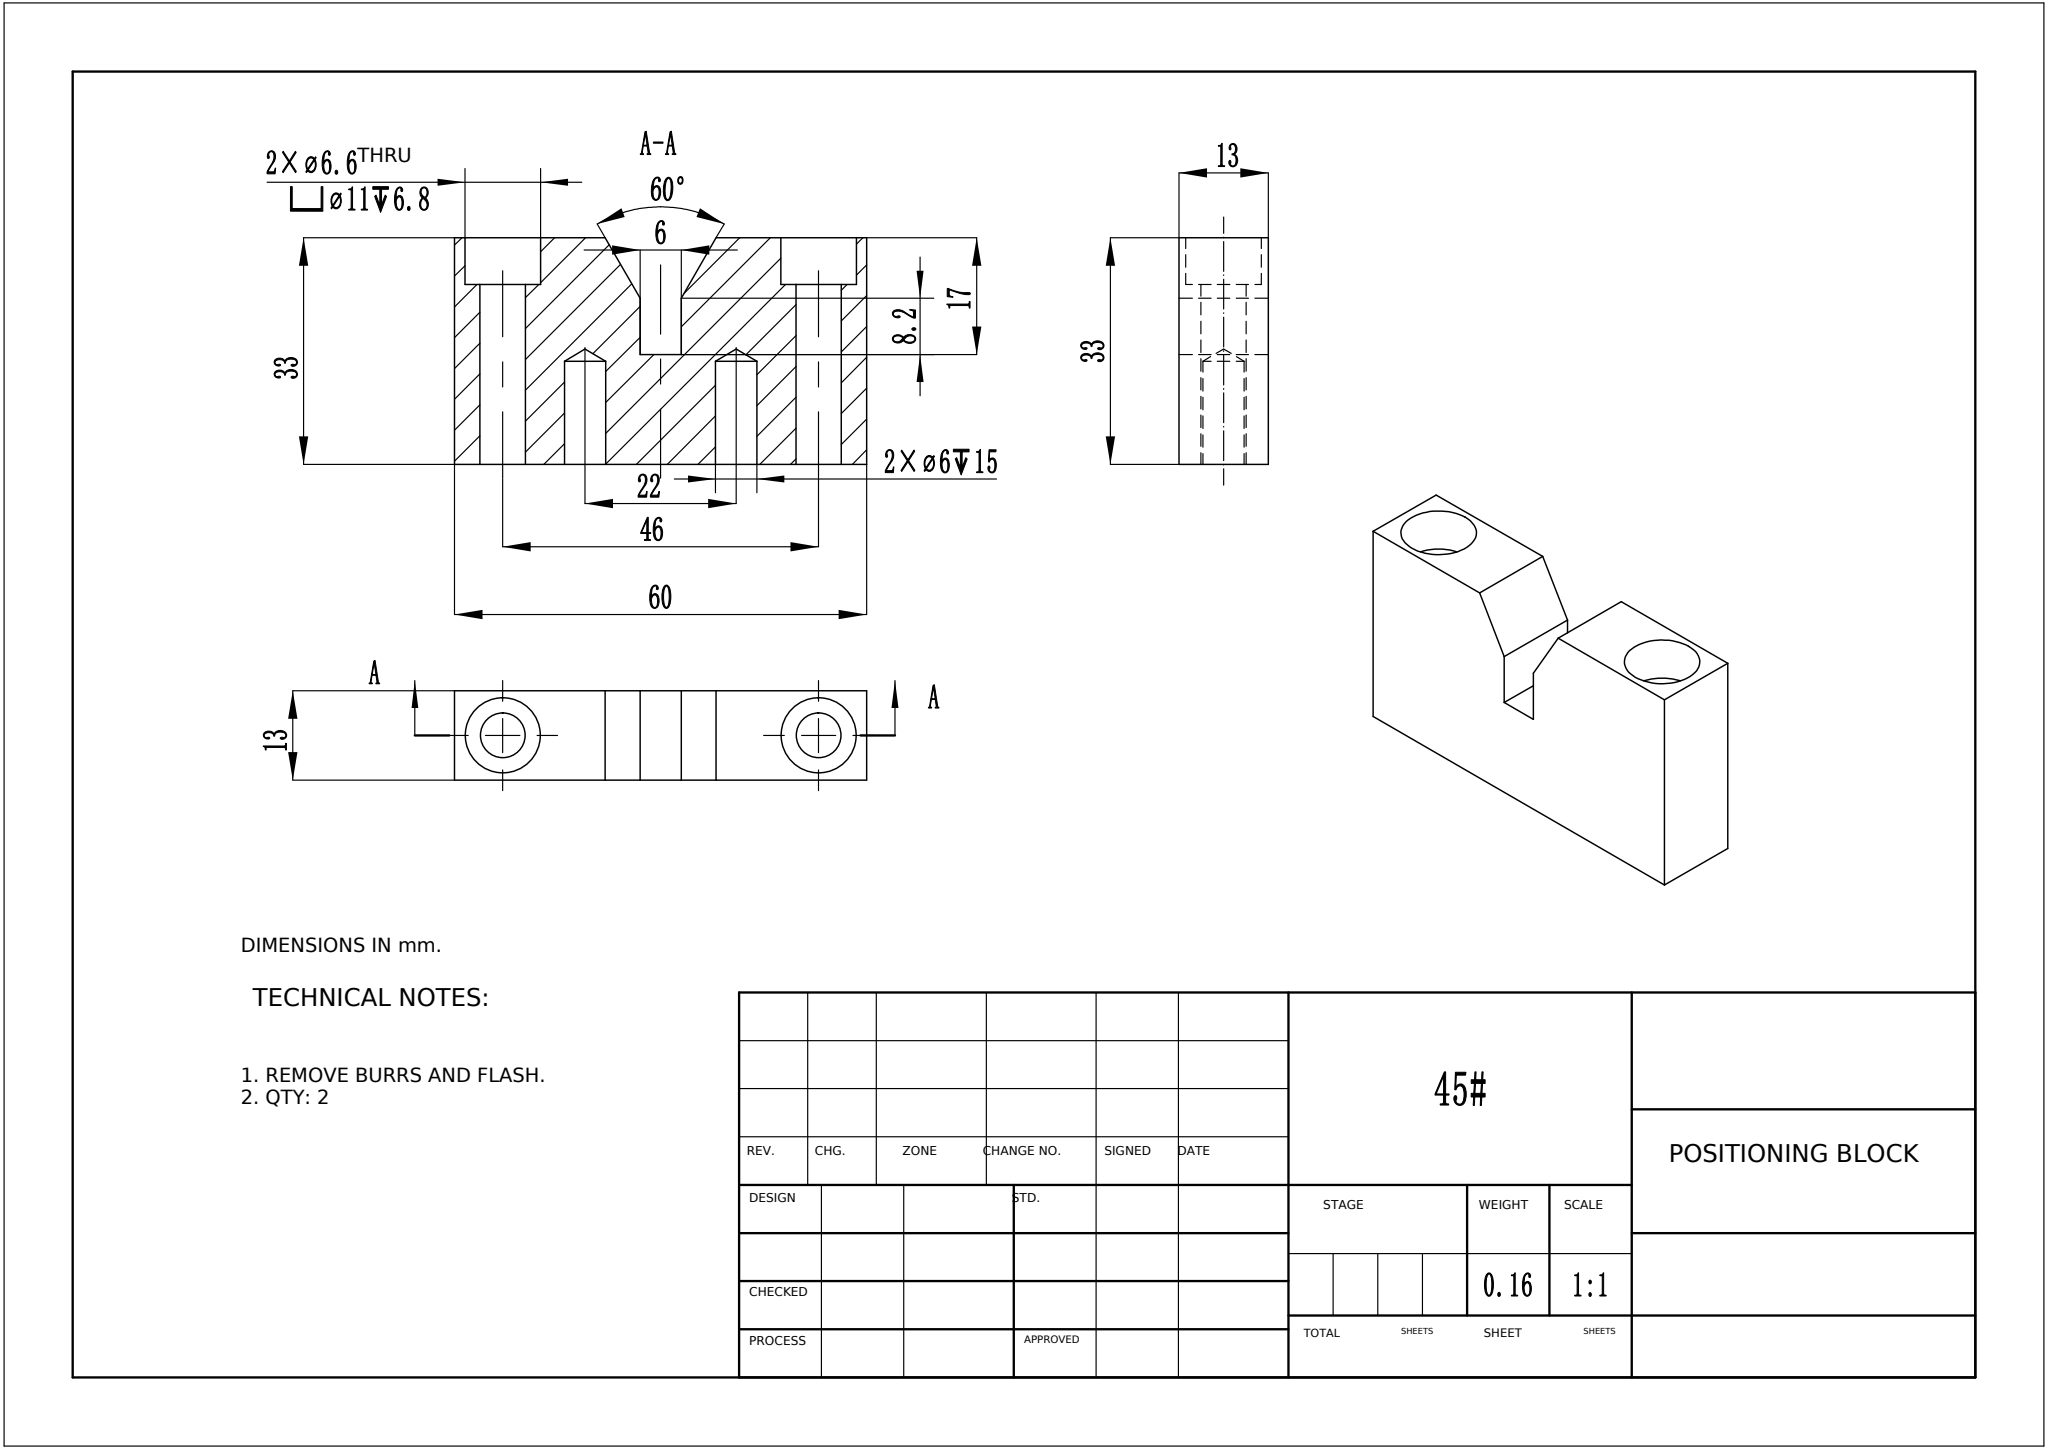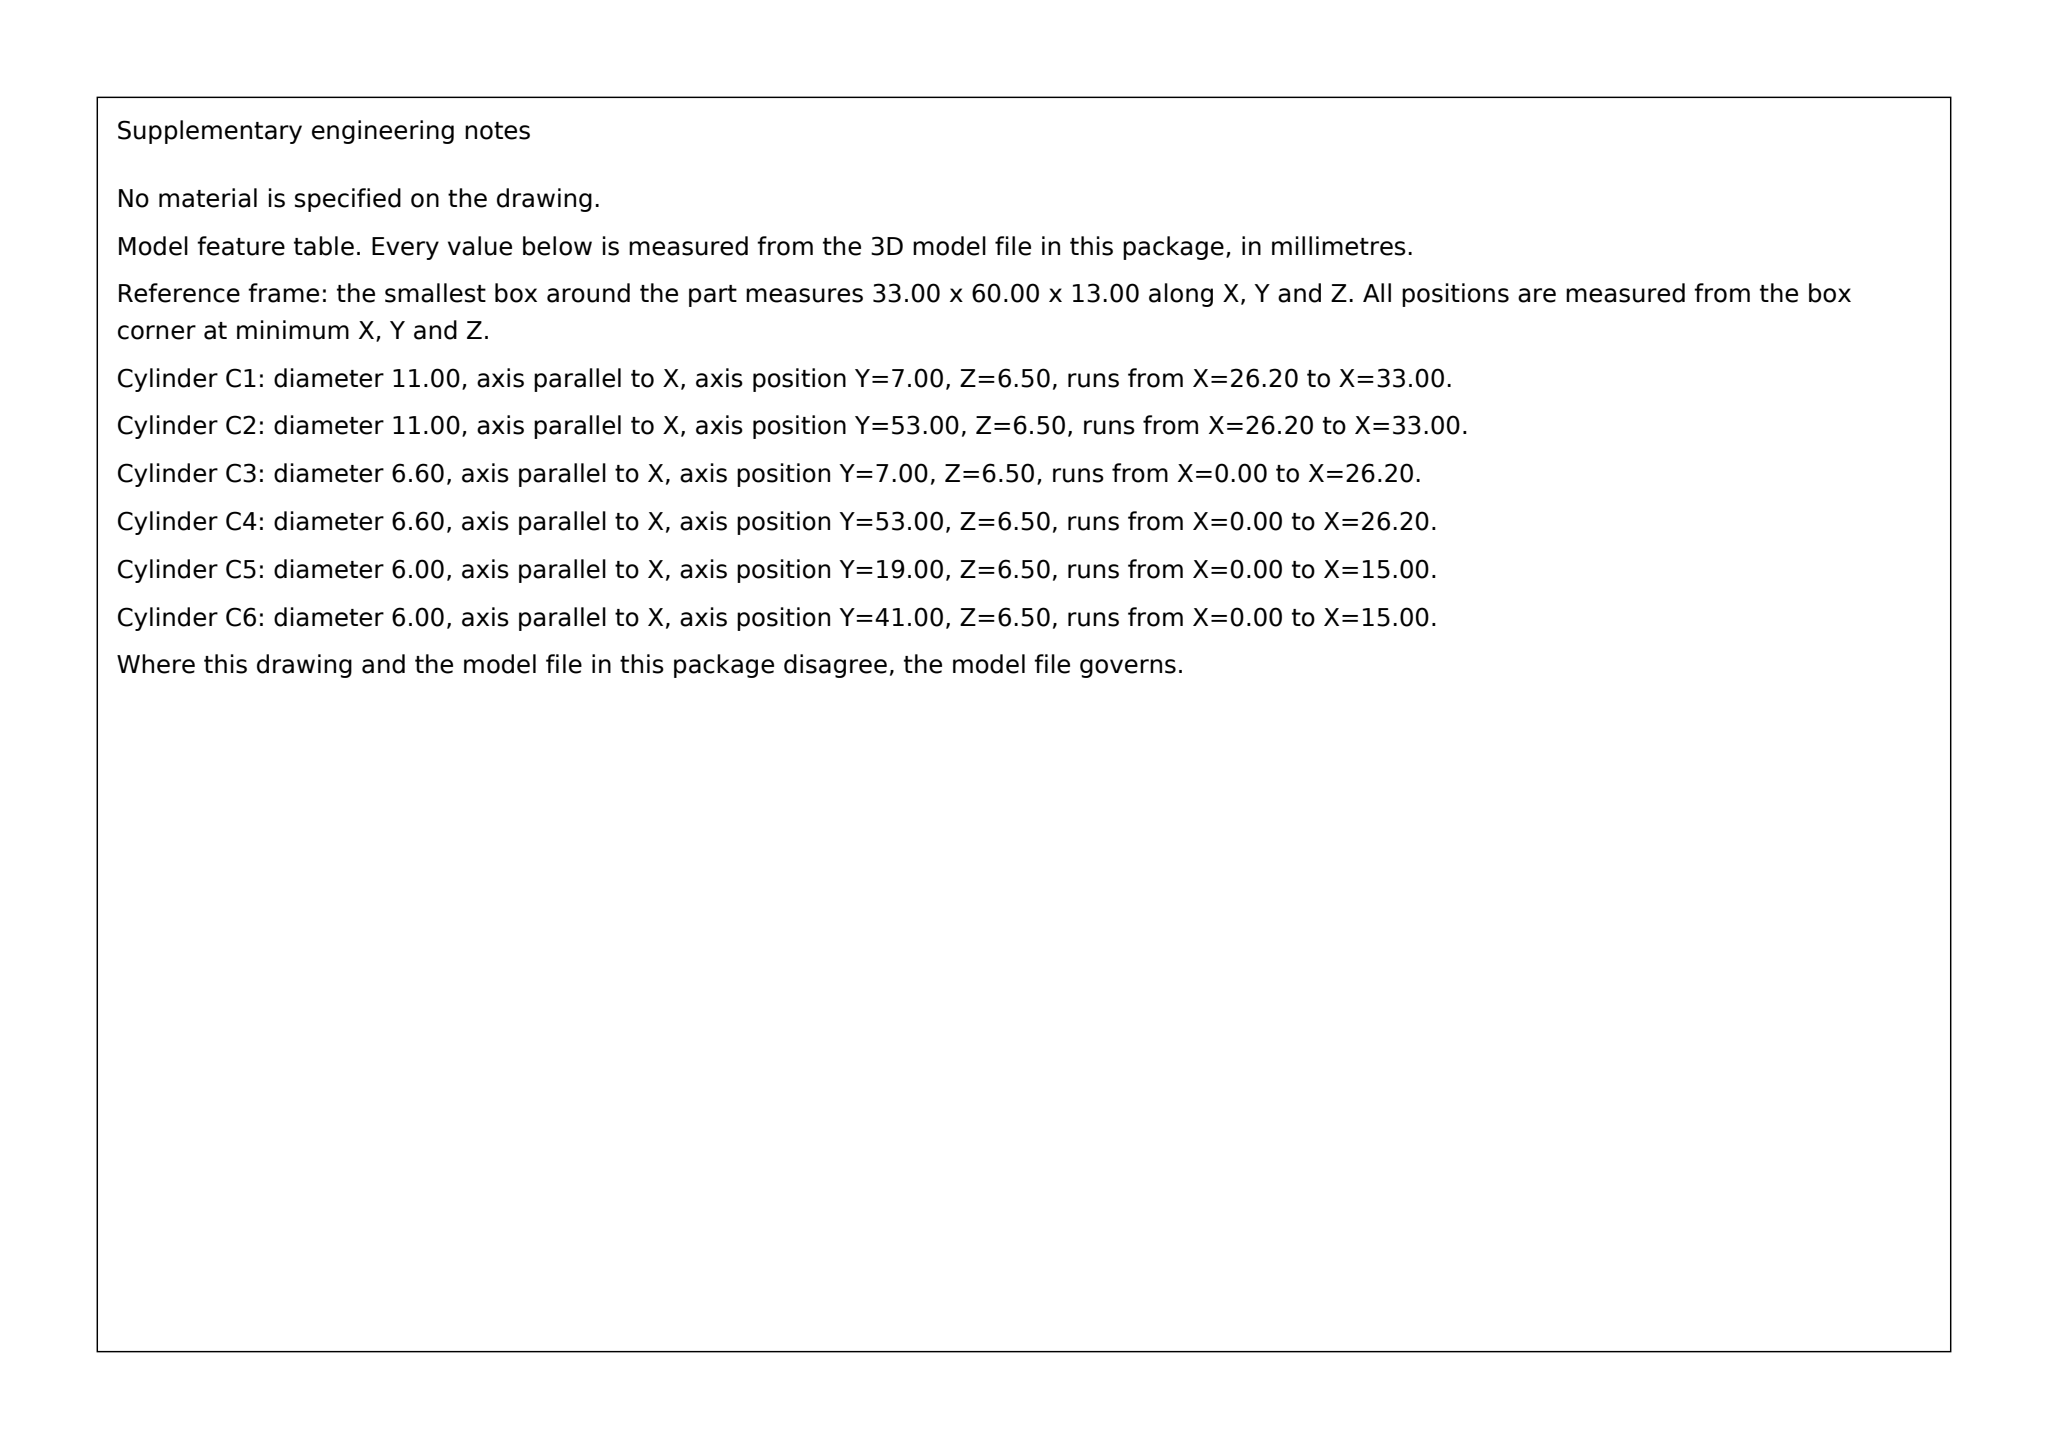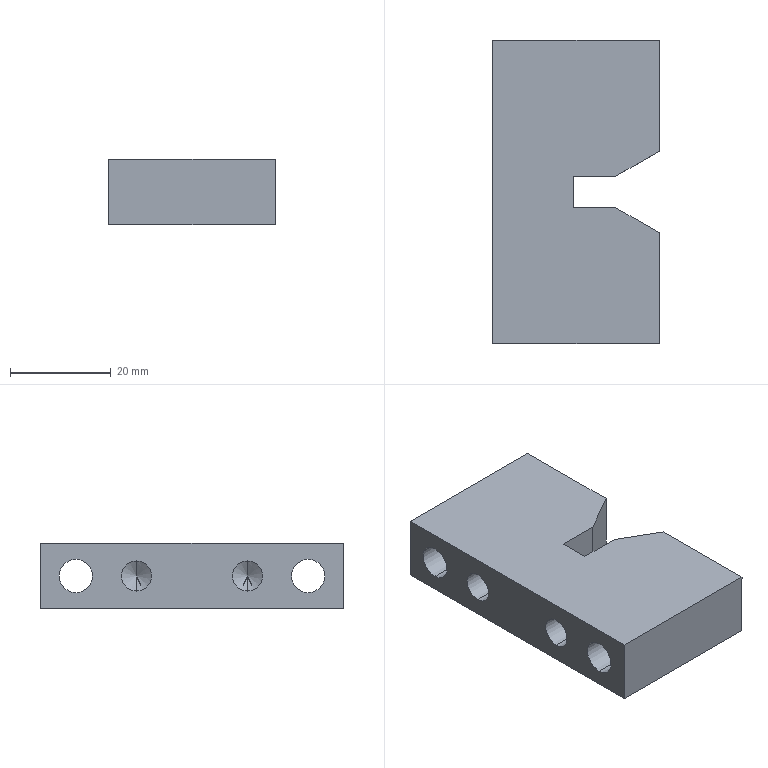Part | SolidWorks | mm | 1 solid | 30 faces | box 33 x 60 x 13 mm | volume 19865 mm3 | plane 14 | cylinder 12 | cone 4 | commonest cylinder face diameters 6 x4 11 x4 6.6 x4
build123d program:
from build123d import *

# Parameters (mm, degrees)
SKETCH1_W                                       = 100
SKETCH1_H                                       = 60
BOSS_EXTRUDE1_DEPTH                             = 50
SKETCH3_R                                       = 6.75
CUT_EXTRUDE1_DEPTH                              = 116.758
BOSS_EXTRUDE2_DEPTH                             = 156
CUT_EXTRUDE4_DEPTH                              = 180.818
SKETCH6_W                                       = 65
SKETCH6_H                                       = 60
CUT_EXTRUDE5_DEPTH                              = 63.682
BOSS_EXTRUDE4_DEPTH                             = 13
SKETCH9_W                                       = 13.769
SKETCH9_H                                       = 6
CUT_EXTRUDE6_DEPTH                              = 52.517
MOVE_FACE1_BY                                   = 10
SKETCH14_W                                      = 23.752
SKETCH14_H                                      = 71.896
CUT_EXTRUDE9_DEPTH                              = 68
M6_HEX_SOCKET_HEAD_CAP_SCREW_CBORE1_D           = 6.6
M6_HEX_SOCKET_HEAD_CAP_SCREW_CBORE1_CBORE_D     = 11
M6_HEX_SOCKET_HEAD_CAP_SCREW_CBORE1_CBORE_DEPTH = 6.8
F_6_0MM_BLIND_PIN_HOLE1_D                       = 6
F_6_0MM_BLIND_PIN_HOLE1_DEPTH                   = 15
F_6_0MM_BLIND_PIN_HOLE1_TIP                     = 1.803


with BuildPart() as part:
    # Sketch1 → Boss-Extrude1 (new body)
    with BuildSketch(Plane(origin=(0, 0, 0), x_dir=(0, 0, -1), z_dir=(1, 0, 0))):
        Rectangle(SKETCH1_W, SKETCH1_H)
    extrude(amount=BOSS_EXTRUDE1_DEPTH)

    # Sketch3 → Cut-Extrude1 (cut, through all)
    with BuildSketch(Plane.XY.offset(50)):
        with Locations((20, 0)):
            Circle(SKETCH3_R)
    extrude(amount=-CUT_EXTRUDE1_DEPTH, mode=Mode.SUBTRACT)

    # Sketch4 → Boss-Extrude2 (add)
    with BuildSketch(Plane.XY.offset(50)):
        Polygon((6.5, 0), (23, -9.526), (23, -55.864), (61.54, -55.864), (61.54, 64.895), (23, 64.895), (23, 9.526), align=None)
    extrude(amount=-BOSS_EXTRUDE2_DEPTH)

    # Sketch5 → Cut-Extrude4 (cut, through all)
    with BuildSketch(Plane(origin=(0, 0, -106), x_dir=(-1, 0, 0), z_dir=(0, 0, -1))):
        Polygon((-23, 9.526), (-23, 64.895), (-61.54, 64.895), (-61.54, -55.864), (-23, -55.864), (-23, -9.526), (-6.5, 0), align=None)
    extrude(amount=-CUT_EXTRUDE4_DEPTH, mode=Mode.SUBTRACT)

    # Sketch6 → Cut-Extrude5 (cut, through all)
    with BuildSketch(Plane(origin=(23, 0, 0), x_dir=(0, 0, -1), z_dir=(1, 0, 0))):
        with Locations((17.5, 0)):
            Rectangle(SKETCH6_W, SKETCH6_H)
    extrude(amount=-CUT_EXTRUDE5_DEPTH, mode=Mode.SUBTRACT)

    # Sketch10 → Boss-Extrude4 (add)
    with BuildSketch(Plane.XY.offset(50)):
        Polygon((23, 8.083), (9, 0), (23, -8.083), (23, -13.063), (5.064, -13.063), (5.064, 13.423), (23, 13.423), align=None)
    extrude(amount=-BOSS_EXTRUDE4_DEPTH)

    # Sketch9 → Cut-Extrude6 (cut, through all)
    with BuildSketch(Plane.XY.offset(50)):
        with Locations((12.884, 0)):
            Rectangle(SKETCH9_W, SKETCH9_H)
    extrude(amount=-CUT_EXTRUDE6_DEPTH, mode=Mode.SUBTRACT)

    # Move Face1: a face moved outward by 10.0
    extrude(part.faces().sort_by_distance((0, 0, 32.5))[0], amount=MOVE_FACE1_BY, dir=(-1, 0, 0))

    # Sketch14 → Cut-Extrude9 (cut, through all)
    with BuildSketch(Plane(origin=(23, 0, 0), x_dir=(0, 0, -1), z_dir=(1, 0, 0))):
        with Locations((-25.124, 2.799)):
            Rectangle(SKETCH14_W, SKETCH14_H)
    extrude(amount=-CUT_EXTRUDE9_DEPTH, mode=Mode.SUBTRACT)

    # M6 Hex Socket Head Cap Screw CBORE1 (through all)
    with Locations(Plane(origin=(23, 0, 0), x_dir=(0, 0, -1), z_dir=(1, 0, 0))):
        with Locations((-43.5, 23), (-43.5, -23)):
            CounterBoreHole(M6_HEX_SOCKET_HEAD_CAP_SCREW_CBORE1_D / 2, M6_HEX_SOCKET_HEAD_CAP_SCREW_CBORE1_CBORE_D / 2, M6_HEX_SOCKET_HEAD_CAP_SCREW_CBORE1_CBORE_DEPTH)

    # 6.0mm Blind Pin Hole1
    with Locations(Plane.ZY.offset(10)):
        with Locations((43.5, 11), (43.5, -11)):
            Hole(F_6_0MM_BLIND_PIN_HOLE1_D / 2, depth=F_6_0MM_BLIND_PIN_HOLE1_DEPTH)
            with Locations((0, 0, -(F_6_0MM_BLIND_PIN_HOLE1_DEPTH + F_6_0MM_BLIND_PIN_HOLE1_TIP / 2))):  # 118° drill point
                Cone(0, F_6_0MM_BLIND_PIN_HOLE1_D / 2, F_6_0MM_BLIND_PIN_HOLE1_TIP, mode=Mode.SUBTRACT)


solid = part.part
STEP:
#1=CARTESIAN_POINT('',(5.,11.,40.5));
#2=VERTEX_POINT('',#1);
#3=CARTESIAN_POINT('',(5.,11.,46.5));
#4=VERTEX_POINT('',#3);
#5=CARTESIAN_POINT('',(5.,11.,43.5));
#6=DIRECTION('',(-1.,0.,0.));
#7=DIRECTION('',(0.,0.,1.));
#8=AXIS2_PLACEMENT_3D('',#5,#6,#7);
#9=CIRCLE('',#8,3.);
#10=EDGE_CURVE('',#2,#4,#9,.T.);
#11=ORIENTED_EDGE('',*,*,#10,.F.);
#12=CARTESIAN_POINT('',(-10.,11.,40.5));
#13=VERTEX_POINT('',#12);
#14=CARTESIAN_POINT('',(-10.,11.,40.5));
#15=DIRECTION('',(-1.,0.,0.));
#16=VECTOR('',#15,1000.);
#17=LINE('',#14,#16);
#18=EDGE_CURVE('',#2,#13,#17,.T.);
#19=ORIENTED_EDGE('',*,*,#18,.T.);
#20=CARTESIAN_POINT('',(-10.,11.,46.5));
#21=VERTEX_POINT('',#20);
#22=CARTESIAN_POINT('',(-10.,11.,43.5));
#23=DIRECTION('',(-1.,0.,0.));
#24=DIRECTION('',(0.,0.,1.));
#25=AXIS2_PLACEMENT_3D('',#22,#23,#24);
#26=CIRCLE('',#25,3.);
#27=EDGE_CURVE('',#13,#21,#26,.T.);
#28=ORIENTED_EDGE('',*,*,#27,.T.);
#29=CARTESIAN_POINT('',(-10.,11.,46.5));
#30=DIRECTION('',(-1.,0.,0.));
#31=VECTOR('',#30,1000.);
#32=LINE('',#29,#31);
#33=EDGE_CURVE('',#4,#21,#32,.T.);
#34=ORIENTED_EDGE('',*,*,#33,.F.);
#35=EDGE_LOOP('',(#11,#19,#28,#34));
#36=FACE_OUTER_BOUND('',#35,.T.);
#37=CARTESIAN_POINT('',(-10.,11.,43.5));
#38=DIRECTION('',(-1.,0.,0.));
#39=DIRECTION('',(0.,0.,1.));
#40=AXIS2_PLACEMENT_3D('',#37,#38,#39);
#41=CYLINDRICAL_SURFACE('',#40,3.);
#42=ADVANCED_FACE('',(#36),#41,.F.);
#43=CARTESIAN_POINT('',(6.803,11.,43.5));
#44=VERTEX_POINT('',#43);
#45=CARTESIAN_POINT('',(5.,11.,46.5));
#46=DIRECTION('',(-0.515,0.,0.8572));
#47=VECTOR('',#46,1000.);
#48=LINE('',#45,#47);
#49=EDGE_CURVE('',#44,#4,#48,.T.);
#50=ORIENTED_EDGE('',*,*,#49,.F.);
#51=CARTESIAN_POINT('',(5.,11.,40.5));
#52=DIRECTION('',(-0.515,0.,-0.8572));
#53=VECTOR('',#52,1000.);
#54=LINE('',#51,#53);
#55=EDGE_CURVE('',#44,#2,#54,.T.);
#56=ORIENTED_EDGE('',*,*,#55,.T.);
#57=ORIENTED_EDGE('',*,*,#10,.T.);
#58=EDGE_LOOP('',(#50,#56,#57));
#59=FACE_OUTER_BOUND('',#58,.T.);
#60=CARTESIAN_POINT('',(5.,11.,43.5));
#61=DIRECTION('',(-1.,0.,0.));
#62=DIRECTION('',(0.,0.,1.));
#63=AXIS2_PLACEMENT_3D('',#60,#61,#62);
#64=CONICAL_SURFACE('',#63,3.,1.03);
#65=ADVANCED_FACE('',(#59),#64,.F.);
#66=CARTESIAN_POINT('',(5.,-11.,40.5));
#67=VERTEX_POINT('',#66);
#68=CARTESIAN_POINT('',(5.,-11.,46.5));
#69=VERTEX_POINT('',#68);
#70=CARTESIAN_POINT('',(5.,-11.,43.5));
#71=DIRECTION('',(-1.,0.,0.));
#72=DIRECTION('',(0.,0.,1.));
#73=AXIS2_PLACEMENT_3D('',#70,#71,#72);
#74=CIRCLE('',#73,3.);
#75=EDGE_CURVE('',#67,#69,#74,.T.);
#76=ORIENTED_EDGE('',*,*,#75,.F.);
#77=CARTESIAN_POINT('',(-10.,-11.,40.5));
#78=VERTEX_POINT('',#77);
#79=CARTESIAN_POINT('',(-10.,-11.,40.5));
#80=DIRECTION('',(-1.,0.,0.));
#81=VECTOR('',#80,1000.);
#82=LINE('',#79,#81);
#83=EDGE_CURVE('',#67,#78,#82,.T.);
#84=ORIENTED_EDGE('',*,*,#83,.T.);
#85=CARTESIAN_POINT('',(-10.,-11.,46.5));
#86=VERTEX_POINT('',#85);
#87=CARTESIAN_POINT('',(-10.,-11.,43.5));
#88=DIRECTION('',(-1.,0.,0.));
#89=DIRECTION('',(0.,0.,1.));
#90=AXIS2_PLACEMENT_3D('',#87,#88,#89);
#91=CIRCLE('',#90,3.);
#92=EDGE_CURVE('',#78,#86,#91,.T.);
#93=ORIENTED_EDGE('',*,*,#92,.T.);
#94=CARTESIAN_POINT('',(-10.,-11.,46.5));
#95=DIRECTION('',(-1.,0.,0.));
#96=VECTOR('',#95,1000.);
#97=LINE('',#94,#96);
#98=EDGE_CURVE('',#69,#86,#97,.T.);
#99=ORIENTED_EDGE('',*,*,#98,.F.);
#100=EDGE_LOOP('',(#76,#84,#93,#99));
#101=FACE_OUTER_BOUND('',#100,.T.);
#102=CARTESIAN_POINT('',(-10.,-11.,43.5));
#103=DIRECTION('',(-1.,0.,0.));
#104=DIRECTION('',(0.,0.,1.));
#105=AXIS2_PLACEMENT_3D('',#102,#103,#104);
#106=CYLINDRICAL_SURFACE('',#105,3.);
#107=ADVANCED_FACE('',(#101),#106,.F.);
#108=CARTESIAN_POINT('',(6.803,-11.,43.5));
#109=VERTEX_POINT('',#108);
#110=CARTESIAN_POINT('',(5.,-11.,46.5));
#111=DIRECTION('',(-0.515,0.,0.8572));
#112=VECTOR('',#111,1000.);
#113=LINE('',#110,#112);
#114=EDGE_CURVE('',#109,#69,#113,.T.);
#115=ORIENTED_EDGE('',*,*,#114,.F.);
#116=CARTESIAN_POINT('',(5.,-11.,40.5));
#117=DIRECTION('',(-0.515,0.,-0.8572));
#118=VECTOR('',#117,1000.);
#119=LINE('',#116,#118);
#120=EDGE_CURVE('',#109,#67,#119,.T.);
#121=ORIENTED_EDGE('',*,*,#120,.T.);
#122=ORIENTED_EDGE('',*,*,#75,.T.);
#123=EDGE_LOOP('',(#115,#121,#122));
#124=FACE_OUTER_BOUND('',#123,.T.);
#125=CARTESIAN_POINT('',(5.,-11.,43.5));
#126=DIRECTION('',(-1.,0.,0.));
#127=DIRECTION('',(0.,0.,1.));
#128=AXIS2_PLACEMENT_3D('',#125,#126,#127);
#129=CONICAL_SURFACE('',#128,3.,1.03);
#130=ADVANCED_FACE('',(#124),#129,.F.);
#131=CARTESIAN_POINT('',(16.2,23.,49.));
#132=VERTEX_POINT('',#131);
#133=CARTESIAN_POINT('',(16.2,23.,38.));
#134=VERTEX_POINT('',#133);
#135=CARTESIAN_POINT('',(16.2,23.,43.5));
#136=DIRECTION('',(1.,0.,0.));
#137=DIRECTION('',(0.,0.,-1.));
#138=AXIS2_PLACEMENT_3D('',#135,#136,#137);
#139=CIRCLE('',#138,5.5);
#140=EDGE_CURVE('',#132,#134,#139,.T.);
#141=ORIENTED_EDGE('',*,*,#140,.F.);
#142=CARTESIAN_POINT('',(23.,23.,49.));
#143=VERTEX_POINT('',#142);
#144=CARTESIAN_POINT('',(23.,23.,49.));
#145=DIRECTION('',(1.,0.,0.));
#146=VECTOR('',#145,1000.);
#147=LINE('',#144,#146);
#148=EDGE_CURVE('',#132,#143,#147,.T.);
#149=ORIENTED_EDGE('',*,*,#148,.T.);
#150=CARTESIAN_POINT('',(23.,23.,38.));
#151=VERTEX_POINT('',#150);
#152=CARTESIAN_POINT('',(23.,23.,43.5));
#153=DIRECTION('',(1.,0.,0.));
#154=DIRECTION('',(0.,0.,-1.));
#155=AXIS2_PLACEMENT_3D('',#152,#153,#154);
#156=CIRCLE('',#155,5.5);
#157=EDGE_CURVE('',#143,#151,#156,.T.);
#158=ORIENTED_EDGE('',*,*,#157,.T.);
#159=CARTESIAN_POINT('',(23.,23.,38.));
#160=DIRECTION('',(1.,0.,0.));
#161=VECTOR('',#160,1000.);
#162=LINE('',#159,#161);
#163=EDGE_CURVE('',#134,#151,#162,.T.);
#164=ORIENTED_EDGE('',*,*,#163,.F.);
#165=EDGE_LOOP('',(#141,#149,#158,#164));
#166=FACE_OUTER_BOUND('',#165,.T.);
#167=CARTESIAN_POINT('',(23.,23.,43.5));
#168=DIRECTION('',(1.,0.,0.));
#169=DIRECTION('',(0.,0.,-1.));
#170=AXIS2_PLACEMENT_3D('',#167,#168,#169);
#171=CYLINDRICAL_SURFACE('',#170,5.5);
#172=ADVANCED_FACE('',(#166),#171,.F.);
#173=CARTESIAN_POINT('',(-10.,23.,46.8));
#174=VERTEX_POINT('',#173);
#175=CARTESIAN_POINT('',(-10.,23.,40.2));
#176=VERTEX_POINT('',#175);
#177=CARTESIAN_POINT('',(-10.,23.,43.5));
#178=DIRECTION('',(1.,0.,0.));
#179=DIRECTION('',(0.,0.,-1.));
#180=AXIS2_PLACEMENT_3D('',#177,#178,#179);
#181=CIRCLE('',#180,3.3);
#182=EDGE_CURVE('',#174,#176,#181,.T.);
#183=ORIENTED_EDGE('',*,*,#182,.F.);
#184=CARTESIAN_POINT('',(16.2,23.,46.8));
#185=VERTEX_POINT('',#184);
#186=CARTESIAN_POINT('',(23.,23.,46.8));
#187=DIRECTION('',(1.,0.,0.));
#188=VECTOR('',#187,1000.);
#189=LINE('',#186,#188);
#190=EDGE_CURVE('',#174,#185,#189,.T.);
#191=ORIENTED_EDGE('',*,*,#190,.T.);
#192=CARTESIAN_POINT('',(16.2,23.,40.2));
#193=VERTEX_POINT('',#192);
#194=CARTESIAN_POINT('',(16.2,23.,43.5));
#195=DIRECTION('',(1.,0.,0.));
#196=DIRECTION('',(0.,0.,-1.));
#197=AXIS2_PLACEMENT_3D('',#194,#195,#196);
#198=CIRCLE('',#197,3.3);
#199=EDGE_CURVE('',#185,#193,#198,.T.);
#200=ORIENTED_EDGE('',*,*,#199,.T.);
#201=CARTESIAN_POINT('',(23.,23.,40.2));
#202=DIRECTION('',(1.,0.,0.));
#203=VECTOR('',#202,1000.);
#204=LINE('',#201,#203);
#205=EDGE_CURVE('',#176,#193,#204,.T.);
#206=ORIENTED_EDGE('',*,*,#205,.F.);
#207=EDGE_LOOP('',(#183,#191,#200,#206));
#208=FACE_OUTER_BOUND('',#207,.T.);
#209=CARTESIAN_POINT('',(23.,23.,43.5));
#210=DIRECTION('',(1.,0.,0.));
#211=DIRECTION('',(0.,0.,-1.));
#212=AXIS2_PLACEMENT_3D('',#209,#210,#211);
#213=CYLINDRICAL_SURFACE('',#212,3.3);
#214=ADVANCED_FACE('',(#208),#213,.F.);
#215=CARTESIAN_POINT('',(16.2,-23.,49.));
#216=VERTEX_POINT('',#215);
#217=CARTESIAN_POINT('',(16.2,-23.,38.));
#218=VERTEX_POINT('',#217);
#219=CARTESIAN_POINT('',(16.2,-23.,43.5));
#220=DIRECTION('',(1.,0.,0.));
#221=DIRECTION('',(0.,0.,-1.));
#222=AXIS2_PLACEMENT_3D('',#219,#220,#221);
#223=CIRCLE('',#222,5.5);
#224=EDGE_CURVE('',#216,#218,#223,.T.);
#225=ORIENTED_EDGE('',*,*,#224,.F.);
#226=CARTESIAN_POINT('',(23.,-23.,49.));
#227=VERTEX_POINT('',#226);
#228=CARTESIAN_POINT('',(23.,-23.,49.));
#229=DIRECTION('',(1.,0.,0.));
#230=VECTOR('',#229,1000.);
#231=LINE('',#228,#230);
#232=EDGE_CURVE('',#216,#227,#231,.T.);
#233=ORIENTED_EDGE('',*,*,#232,.T.);
#234=CARTESIAN_POINT('',(23.,-23.,38.));
#235=VERTEX_POINT('',#234);
#236=CARTESIAN_POINT('',(23.,-23.,43.5));
#237=DIRECTION('',(1.,0.,0.));
#238=DIRECTION('',(0.,0.,-1.));
#239=AXIS2_PLACEMENT_3D('',#236,#237,#238);
#240=CIRCLE('',#239,5.5);
#241=EDGE_CURVE('',#227,#235,#240,.T.);
#242=ORIENTED_EDGE('',*,*,#241,.T.);
#243=CARTESIAN_POINT('',(23.,-23.,38.));
#244=DIRECTION('',(1.,0.,0.));
#245=VECTOR('',#244,1000.);
#246=LINE('',#243,#245);
#247=EDGE_CURVE('',#218,#235,#246,.T.);
#248=ORIENTED_EDGE('',*,*,#247,.F.);
#249=EDGE_LOOP('',(#225,#233,#242,#248));
#250=FACE_OUTER_BOUND('',#249,.T.);
#251=CARTESIAN_POINT('',(23.,-23.,43.5));
#252=DIRECTION('',(1.,0.,0.));
#253=DIRECTION('',(0.,0.,-1.));
#254=AXIS2_PLACEMENT_3D('',#251,#252,#253);
#255=CYLINDRICAL_SURFACE('',#254,5.5);
#256=ADVANCED_FACE('',(#250),#255,.F.);
#257=CARTESIAN_POINT('',(-10.,-23.,46.8));
#258=VERTEX_POINT('',#257);
#259=CARTESIAN_POINT('',(-10.,-23.,40.2));
#260=VERTEX_POINT('',#259);
#261=CARTESIAN_POINT('',(-10.,-23.,43.5));
#262=DIRECTION('',(1.,0.,0.));
#263=DIRECTION('',(0.,0.,-1.));
#264=AXIS2_PLACEMENT_3D('',#261,#262,#263);
#265=CIRCLE('',#264,3.3);
#266=EDGE_CURVE('',#258,#260,#265,.T.);
#267=ORIENTED_EDGE('',*,*,#266,.F.);
#268=CARTESIAN_POINT('',(16.2,-23.,46.8));
#269=VERTEX_POINT('',#268);
#270=CARTESIAN_POINT('',(23.,-23.,46.8));
#271=DIRECTION('',(1.,0.,0.));
#272=VECTOR('',#271,1000.);
#273=LINE('',#270,#272);
#274=EDGE_CURVE('',#258,#269,#273,.T.);
#275=ORIENTED_EDGE('',*,*,#274,.T.);
#276=CARTESIAN_POINT('',(16.2,-23.,40.2));
#277=VERTEX_POINT('',#276);
#278=CARTESIAN_POINT('',(16.2,-23.,43.5));
#279=DIRECTION('',(1.,0.,0.));
#280=DIRECTION('',(0.,0.,-1.));
#281=AXIS2_PLACEMENT_3D('',#278,#279,#280);
#282=CIRCLE('',#281,3.3);
#283=EDGE_CURVE('',#269,#277,#282,.T.);
#284=ORIENTED_EDGE('',*,*,#283,.T.);
#285=CARTESIAN_POINT('',(23.,-23.,40.2));
#286=DIRECTION('',(1.,0.,0.));
#287=VECTOR('',#286,1000.);
#288=LINE('',#285,#287);
#289=EDGE_CURVE('',#260,#277,#288,.T.);
#290=ORIENTED_EDGE('',*,*,#289,.F.);
#291=EDGE_LOOP('',(#267,#275,#284,#290));
#292=FACE_OUTER_BOUND('',#291,.T.);
#293=CARTESIAN_POINT('',(23.,-23.,43.5));
#294=DIRECTION('',(1.,0.,0.));
#295=DIRECTION('',(0.,0.,-1.));
#296=AXIS2_PLACEMENT_3D('',#293,#294,#295);
#297=CYLINDRICAL_SURFACE('',#296,3.3);
#298=ADVANCED_FACE('',(#292),#297,.F.);
#299=CARTESIAN_POINT('',(23.,30.,37.));
#300=VERTEX_POINT('',#299);
#301=CARTESIAN_POINT('',(23.,30.,50.));
#302=VERTEX_POINT('',#301);
#303=CARTESIAN_POINT('',(23.,30.,-50.));
#304=DIRECTION('',(0.,-0.,1.));
#305=VECTOR('',#304,1000.);
#306=LINE('',#303,#305);
#307=EDGE_CURVE('',#300,#302,#306,.T.);
#308=ORIENTED_EDGE('',*,*,#307,.F.);
#309=CARTESIAN_POINT('',(-10.,30.,37.));
#310=VERTEX_POINT('',#309);
#311=CARTESIAN_POINT('',(50.,30.,37.));
#312=DIRECTION('',(-1.,0.,0.));
#313=VECTOR('',#312,1000.);
#314=LINE('',#311,#313);
#315=EDGE_CURVE('',#300,#310,#314,.T.);
#316=ORIENTED_EDGE('',*,*,#315,.T.);
#317=CARTESIAN_POINT('',(-10.,30.,50.));
#318=VERTEX_POINT('',#317);
#319=CARTESIAN_POINT('',(-10.,30.,-50.));
#320=DIRECTION('',(0.,-0.,1.));
#321=VECTOR('',#320,1000.);
#322=LINE('',#319,#321);
#323=EDGE_CURVE('',#310,#318,#322,.T.);
#324=ORIENTED_EDGE('',*,*,#323,.T.);
#325=CARTESIAN_POINT('',(50.,30.,50.));
#326=DIRECTION('',(-1.,0.,0.));
#327=VECTOR('',#326,1000.);
#328=LINE('',#325,#327);
#329=EDGE_CURVE('',#302,#318,#328,.T.);
#330=ORIENTED_EDGE('',*,*,#329,.F.);
#331=EDGE_LOOP('',(#308,#316,#324,#330));
#332=FACE_OUTER_BOUND('',#331,.T.);
#333=CARTESIAN_POINT('',(50.,30.,-50.));
#334=DIRECTION('',(0.,-1.,-0.));
#335=DIRECTION('',(0.,0.,-1.));
#336=AXIS2_PLACEMENT_3D('',#333,#334,#335);
#337=PLANE('',#336);
#338=ADVANCED_FACE('',(#332),#337,.F.);
#339=CARTESIAN_POINT('',(6.,3.,50.));
#340=VERTEX_POINT('',#339);
#341=CARTESIAN_POINT('',(6.,-3.,50.));
#342=VERTEX_POINT('',#341);
#343=CARTESIAN_POINT('',(6.,-3.,50.));
#344=DIRECTION('',(0.,-1.,0.));
#345=VECTOR('',#344,1000.);
#346=LINE('',#343,#345);
#347=EDGE_CURVE('',#340,#342,#346,.T.);
#348=ORIENTED_EDGE('',*,*,#347,.F.);
#349=CARTESIAN_POINT('',(14.196,3.,50.));
#350=VERTEX_POINT('',#349);
#351=CARTESIAN_POINT('',(19.769,3.,50.));
#352=DIRECTION('',(-1.,-0.,0.));
#353=VECTOR('',#352,1000.);
#354=LINE('',#351,#353);
#355=EDGE_CURVE('',#350,#340,#354,.T.);
#356=ORIENTED_EDGE('',*,*,#355,.F.);
#357=CARTESIAN_POINT('',(23.,8.083,50.));
#358=VERTEX_POINT('',#357);
#359=CARTESIAN_POINT('',(23.,8.083,50.));
#360=DIRECTION('',(0.866,0.5,0.));
#361=VECTOR('',#360,1000.);
#362=LINE('',#359,#361);
#363=EDGE_CURVE('',#350,#358,#362,.T.);
#364=ORIENTED_EDGE('',*,*,#363,.T.);
#365=CARTESIAN_POINT('',(23.,9.526,50.));
#366=DIRECTION('',(0.,1.,0.));
#367=VECTOR('',#366,1000.);
#368=LINE('',#365,#367);
#369=EDGE_CURVE('',#358,#302,#368,.T.);
#370=ORIENTED_EDGE('',*,*,#369,.T.);
#371=ORIENTED_EDGE('',*,*,#329,.T.);
#372=CARTESIAN_POINT('',(-10.,-30.,50.));
#373=VERTEX_POINT('',#372);
#374=CARTESIAN_POINT('',(-10.,-30.,50.));
#375=DIRECTION('',(0.,-1.,0.));
#376=VECTOR('',#375,1000.);
#377=LINE('',#374,#376);
#378=EDGE_CURVE('',#318,#373,#377,.T.);
#379=ORIENTED_EDGE('',*,*,#378,.T.);
#380=CARTESIAN_POINT('',(23.,-30.,50.));
#381=VERTEX_POINT('',#380);
#382=CARTESIAN_POINT('',(50.,-30.,50.));
#383=DIRECTION('',(-1.,0.,0.));
#384=VECTOR('',#383,1000.);
#385=LINE('',#382,#384);
#386=EDGE_CURVE('',#381,#373,#385,.T.);
#387=ORIENTED_EDGE('',*,*,#386,.F.);
#388=CARTESIAN_POINT('',(23.,-8.083,50.));
#389=VERTEX_POINT('',#388);
#390=CARTESIAN_POINT('',(23.,-55.864,50.));
#391=DIRECTION('',(0.,1.,0.));
#392=VECTOR('',#391,1000.);
#393=LINE('',#390,#392);
#394=EDGE_CURVE('',#381,#389,#393,.T.);
#395=ORIENTED_EDGE('',*,*,#394,.T.);
#396=CARTESIAN_POINT('',(14.196,-3.,50.));
#397=VERTEX_POINT('',#396);
#398=CARTESIAN_POINT('',(23.,-8.083,50.));
#399=DIRECTION('',(-0.866,0.5,0.));
#400=VECTOR('',#399,1000.);
#401=LINE('',#398,#400);
#402=EDGE_CURVE('',#389,#397,#401,.T.);
#403=ORIENTED_EDGE('',*,*,#402,.T.);
#404=CARTESIAN_POINT('',(19.769,-3.,50.));
#405=DIRECTION('',(1.,0.,0.));
#406=VECTOR('',#405,1000.);
#407=LINE('',#404,#406);
#408=EDGE_CURVE('',#342,#397,#407,.T.);
#409=ORIENTED_EDGE('',*,*,#408,.F.);
#410=EDGE_LOOP('',(#348,#356,#364,#370,#371,#379,#387,#395,#403,#409));
#411=FACE_OUTER_BOUND('',#410,.T.);
#412=CARTESIAN_POINT('',(50.,-30.,50.));
#413=DIRECTION('',(0.,0.,-1.));
#414=DIRECTION('',(-1.,0.,0.));
#415=AXIS2_PLACEMENT_3D('',#412,#413,#414);
#416=PLANE('',#415);
#417=ADVANCED_FACE('',(#411),#416,.F.);
#418=CARTESIAN_POINT('',(-10.,-30.,37.));
#419=VERTEX_POINT('',#418);
#420=CARTESIAN_POINT('',(-10.,-30.,-50.));
#421=DIRECTION('',(0.,0.,-1.));
#422=VECTOR('',#421,1000.);
#423=LINE('',#420,#422);
#424=EDGE_CURVE('',#373,#419,#423,.T.);
#425=ORIENTED_EDGE('',*,*,#424,.T.);
#426=CARTESIAN_POINT('',(23.,-30.,37.));
#427=VERTEX_POINT('',#426);
#428=CARTESIAN_POINT('',(50.,-30.,37.));
#429=DIRECTION('',(1.,0.,0.));
#430=VECTOR('',#429,1000.);
#431=LINE('',#428,#430);
#432=EDGE_CURVE('',#419,#427,#431,.T.);
#433=ORIENTED_EDGE('',*,*,#432,.T.);
#434=CARTESIAN_POINT('',(23.,-30.,-50.));
#435=DIRECTION('',(-0.,-0.,1.));
#436=VECTOR('',#435,1000.);
#437=LINE('',#434,#436);
#438=EDGE_CURVE('',#427,#381,#437,.T.);
#439=ORIENTED_EDGE('',*,*,#438,.T.);
#440=ORIENTED_EDGE('',*,*,#386,.T.);
#441=EDGE_LOOP('',(#425,#433,#439,#440));
#442=FACE_OUTER_BOUND('',#441,.T.);
#443=CARTESIAN_POINT('',(50.,-30.,-50.));
#444=DIRECTION('',(0.,1.,0.));
#445=DIRECTION('',(0.,-0.,1.));
#446=AXIS2_PLACEMENT_3D('',#443,#444,#445);
#447=PLANE('',#446);
#448=ADVANCED_FACE('',(#442),#447,.F.);
#449=CARTESIAN_POINT('',(-10.,11.,43.5));
#450=DIRECTION('',(-1.,0.,0.));
#451=DIRECTION('',(0.,0.,1.));
#452=AXIS2_PLACEMENT_3D('',#449,#450,#451);
#453=CIRCLE('',#452,3.);
#454=EDGE_CURVE('',#21,#13,#453,.T.);
#455=ORIENTED_EDGE('',*,*,#454,.F.);
#456=ORIENTED_EDGE('',*,*,#27,.F.);
#457=EDGE_LOOP('',(#455,#456));
#458=FACE_BOUND('',#457,.T.);
#459=CARTESIAN_POINT('',(-10.,-11.,43.5));
#460=DIRECTION('',(-1.,0.,0.));
#461=DIRECTION('',(0.,0.,1.));
#462=AXIS2_PLACEMENT_3D('',#459,#460,#461);
#463=CIRCLE('',#462,3.);
#464=EDGE_CURVE('',#86,#78,#463,.T.);
#465=ORIENTED_EDGE('',*,*,#464,.F.);
#466=ORIENTED_EDGE('',*,*,#92,.F.);
#467=EDGE_LOOP('',(#465,#466));
#468=FACE_BOUND('',#467,.T.);
#469=CARTESIAN_POINT('',(-10.,23.,43.5));
#470=DIRECTION('',(1.,0.,0.));
#471=DIRECTION('',(0.,0.,-1.));
#472=AXIS2_PLACEMENT_3D('',#469,#470,#471);
#473=CIRCLE('',#472,3.3);
#474=EDGE_CURVE('',#176,#174,#473,.T.);
#475=ORIENTED_EDGE('',*,*,#474,.T.);
#476=ORIENTED_EDGE('',*,*,#182,.T.);
#477=EDGE_LOOP('',(#475,#476));
#478=FACE_BOUND('',#477,.T.);
#479=CARTESIAN_POINT('',(-10.,-23.,43.5));
#480=DIRECTION('',(1.,0.,0.));
#481=DIRECTION('',(0.,0.,-1.));
#482=AXIS2_PLACEMENT_3D('',#479,#480,#481);
#483=CIRCLE('',#482,3.3);
#484=EDGE_CURVE('',#260,#258,#483,.T.);
#485=ORIENTED_EDGE('',*,*,#484,.T.);
#486=ORIENTED_EDGE('',*,*,#266,.T.);
#487=EDGE_LOOP('',(#485,#486));
#488=FACE_BOUND('',#487,.T.);
#489=ORIENTED_EDGE('',*,*,#323,.F.);
#490=CARTESIAN_POINT('',(-10.,-33.149,37.));
#491=DIRECTION('',(0.,-1.,0.));
#492=VECTOR('',#491,1000.);
#493=LINE('',#490,#492);
#494=EDGE_CURVE('',#310,#419,#493,.T.);
#495=ORIENTED_EDGE('',*,*,#494,.T.);
#496=ORIENTED_EDGE('',*,*,#424,.F.);
#497=ORIENTED_EDGE('',*,*,#378,.F.);
#498=EDGE_LOOP('',(#489,#495,#496,#497));
#499=FACE_OUTER_BOUND('',#498,.T.);
#500=CARTESIAN_POINT('',(-10.,0.,0.));
#501=DIRECTION('',(1.,0.,0.));
#502=DIRECTION('',(0.,0.,-1.));
#503=AXIS2_PLACEMENT_3D('',#500,#501,#502);
#504=PLANE('',#503);
#505=ADVANCED_FACE('',(#458,#468,#478,#488,#499),#504,.F.);
#506=CARTESIAN_POINT('',(23.,-23.,43.5));
#507=DIRECTION('',(1.,0.,0.));
#508=DIRECTION('',(0.,0.,-1.));
#509=AXIS2_PLACEMENT_3D('',#506,#507,#508);
#510=CIRCLE('',#509,5.5);
#511=EDGE_CURVE('',#235,#227,#510,.T.);
#512=ORIENTED_EDGE('',*,*,#511,.F.);
#513=ORIENTED_EDGE('',*,*,#241,.F.);
#514=EDGE_LOOP('',(#512,#513));
#515=FACE_BOUND('',#514,.T.);
#516=ORIENTED_EDGE('',*,*,#438,.F.);
#517=CARTESIAN_POINT('',(23.,-8.083,37.));
#518=VERTEX_POINT('',#517);
#519=CARTESIAN_POINT('',(23.,-13.063,37.));
#520=DIRECTION('',(0.,1.,0.));
#521=VECTOR('',#520,1000.);
#522=LINE('',#519,#521);
#523=EDGE_CURVE('',#427,#518,#522,.T.);
#524=ORIENTED_EDGE('',*,*,#523,.T.);
#525=CARTESIAN_POINT('',(23.,-8.083,37.));
#526=DIRECTION('',(0.,0.,1.));
#527=VECTOR('',#526,1000.);
#528=LINE('',#525,#527);
#529=EDGE_CURVE('',#518,#389,#528,.T.);
#530=ORIENTED_EDGE('',*,*,#529,.T.);
#531=ORIENTED_EDGE('',*,*,#394,.F.);
#532=EDGE_LOOP('',(#516,#524,#530,#531));
#533=FACE_OUTER_BOUND('',#532,.T.);
#534=CARTESIAN_POINT('',(23.,-55.864,50.));
#535=DIRECTION('',(-1.,0.,0.));
#536=DIRECTION('',(-0.,-1.,0.));
#537=AXIS2_PLACEMENT_3D('',#534,#535,#536);
#538=PLANE('',#537);
#539=ADVANCED_FACE('',(#515,#533),#538,.F.);
#540=CARTESIAN_POINT('',(23.,23.,43.5));
#541=DIRECTION('',(1.,0.,0.));
#542=DIRECTION('',(0.,0.,-1.));
#543=AXIS2_PLACEMENT_3D('',#540,#541,#542);
#544=CIRCLE('',#543,5.5);
#545=EDGE_CURVE('',#151,#143,#544,.T.);
#546=ORIENTED_EDGE('',*,*,#545,.F.);
#547=ORIENTED_EDGE('',*,*,#157,.F.);
#548=EDGE_LOOP('',(#546,#547));
#549=FACE_BOUND('',#548,.T.);
#550=CARTESIAN_POINT('',(23.,8.083,37.));
#551=VERTEX_POINT('',#550);
#552=CARTESIAN_POINT('',(23.,8.083,37.));
#553=DIRECTION('',(-0.,1.,0.));
#554=VECTOR('',#553,1000.);
#555=LINE('',#552,#554);
#556=EDGE_CURVE('',#551,#300,#555,.T.);
#557=ORIENTED_EDGE('',*,*,#556,.T.);
#558=ORIENTED_EDGE('',*,*,#307,.T.);
#559=ORIENTED_EDGE('',*,*,#369,.F.);
#560=CARTESIAN_POINT('',(23.,8.083,37.));
#561=DIRECTION('',(0.,0.,1.));
#562=VECTOR('',#561,1000.);
#563=LINE('',#560,#562);
#564=EDGE_CURVE('',#551,#358,#563,.T.);
#565=ORIENTED_EDGE('',*,*,#564,.F.);
#566=EDGE_LOOP('',(#557,#558,#559,#565));
#567=FACE_OUTER_BOUND('',#566,.T.);
#568=CARTESIAN_POINT('',(23.,9.526,50.));
#569=DIRECTION('',(-1.,0.,0.));
#570=DIRECTION('',(0.,0.,1.));
#571=AXIS2_PLACEMENT_3D('',#568,#569,#570);
#572=PLANE('',#571);
#573=ADVANCED_FACE('',(#549,#567),#572,.F.);
#574=ORIENTED_EDGE('',*,*,#523,.F.);
#575=ORIENTED_EDGE('',*,*,#432,.F.);
#576=ORIENTED_EDGE('',*,*,#494,.F.);
#577=ORIENTED_EDGE('',*,*,#315,.F.);
#578=ORIENTED_EDGE('',*,*,#556,.F.);
#579=CARTESIAN_POINT('',(14.196,3.,37.));
#580=VERTEX_POINT('',#579);
#581=CARTESIAN_POINT('',(23.,8.083,37.));
#582=DIRECTION('',(0.866,0.5,0.));
#583=VECTOR('',#582,1000.);
#584=LINE('',#581,#583);
#585=EDGE_CURVE('',#580,#551,#584,.T.);
#586=ORIENTED_EDGE('',*,*,#585,.F.);
#587=CARTESIAN_POINT('',(6.,3.,37.));
#588=VERTEX_POINT('',#587);
#589=CARTESIAN_POINT('',(-0.,3.,37.));
#590=DIRECTION('',(-1.,-0.,0.));
#591=VECTOR('',#590,1000.);
#592=LINE('',#589,#591);
#593=EDGE_CURVE('',#580,#588,#592,.T.);
#594=ORIENTED_EDGE('',*,*,#593,.T.);
#595=CARTESIAN_POINT('',(6.,-3.,37.));
#596=VERTEX_POINT('',#595);
#597=CARTESIAN_POINT('',(6.,-3.,37.));
#598=DIRECTION('',(0.,1.,0.));
#599=VECTOR('',#598,1000.);
#600=LINE('',#597,#599);
#601=EDGE_CURVE('',#596,#588,#600,.T.);
#602=ORIENTED_EDGE('',*,*,#601,.F.);
#603=CARTESIAN_POINT('',(14.196,-3.,37.));
#604=VERTEX_POINT('',#603);
#605=CARTESIAN_POINT('',(0.,-3.,37.));
#606=DIRECTION('',(1.,0.,0.));
#607=VECTOR('',#606,1000.);
#608=LINE('',#605,#607);
#609=EDGE_CURVE('',#596,#604,#608,.T.);
#610=ORIENTED_EDGE('',*,*,#609,.T.);
#611=CARTESIAN_POINT('',(23.,-8.083,37.));
#612=DIRECTION('',(-0.866,0.5,0.));
#613=VECTOR('',#612,1000.);
#614=LINE('',#611,#613);
#615=EDGE_CURVE('',#518,#604,#614,.T.);
#616=ORIENTED_EDGE('',*,*,#615,.F.);
#617=EDGE_LOOP('',(#574,#575,#576,#577,#578,#586,#594,#602,#610,#616));
#618=FACE_OUTER_BOUND('',#617,.T.);
#619=CARTESIAN_POINT('',(0.,0.,37.));
#620=DIRECTION('',(0.,0.,1.));
#621=DIRECTION('',(1.,0.,0.));
#622=AXIS2_PLACEMENT_3D('',#619,#620,#621);
#623=PLANE('',#622);
#624=ADVANCED_FACE('',(#618),#623,.F.);
#625=CARTESIAN_POINT('',(14.196,3.,37.));
#626=DIRECTION('',(0.,0.,1.));
#627=VECTOR('',#626,1000.);
#628=LINE('',#625,#627);
#629=EDGE_CURVE('',#580,#350,#628,.T.);
#630=ORIENTED_EDGE('',*,*,#629,.F.);
#631=ORIENTED_EDGE('',*,*,#585,.T.);
#632=ORIENTED_EDGE('',*,*,#564,.T.);
#633=ORIENTED_EDGE('',*,*,#363,.F.);
#634=EDGE_LOOP('',(#630,#631,#632,#633));
#635=FACE_OUTER_BOUND('',#634,.T.);
#636=CARTESIAN_POINT('',(23.,8.083,37.));
#637=DIRECTION('',(0.5,-0.866,0.));
#638=DIRECTION('',(0.866,0.5,0.));
#639=AXIS2_PLACEMENT_3D('',#636,#637,#638);
#640=PLANE('',#639);
#641=ADVANCED_FACE('',(#635),#640,.T.);
#642=CARTESIAN_POINT('',(14.196,-3.,37.));
#643=DIRECTION('',(0.,0.,-1.));
#644=VECTOR('',#643,1000.);
#645=LINE('',#642,#644);
#646=EDGE_CURVE('',#397,#604,#645,.T.);
#647=ORIENTED_EDGE('',*,*,#646,.F.);
#648=ORIENTED_EDGE('',*,*,#402,.F.);
#649=ORIENTED_EDGE('',*,*,#529,.F.);
#650=ORIENTED_EDGE('',*,*,#615,.T.);
#651=EDGE_LOOP('',(#647,#648,#649,#650));
#652=FACE_OUTER_BOUND('',#651,.T.);
#653=CARTESIAN_POINT('',(23.,-8.083,37.));
#654=DIRECTION('',(0.5,0.866,0.));
#655=DIRECTION('',(-0.866,0.5,0.));
#656=AXIS2_PLACEMENT_3D('',#653,#654,#655);
#657=PLANE('',#656);
#658=ADVANCED_FACE('',(#652),#657,.T.);
#659=CARTESIAN_POINT('',(6.,3.,15.));
#660=DIRECTION('',(0.,0.,1.));
#661=VECTOR('',#660,1000.);
#662=LINE('',#659,#661);
#663=EDGE_CURVE('',#588,#340,#662,.T.);
#664=ORIENTED_EDGE('',*,*,#663,.F.);
#665=ORIENTED_EDGE('',*,*,#593,.F.);
#666=ORIENTED_EDGE('',*,*,#629,.T.);
#667=ORIENTED_EDGE('',*,*,#355,.T.);
#668=EDGE_LOOP('',(#664,#665,#666,#667));
#669=FACE_OUTER_BOUND('',#668,.T.);
#670=CARTESIAN_POINT('',(19.769,3.,15.));
#671=DIRECTION('',(-0.,1.,0.));
#672=DIRECTION('',(-1.,-0.,0.));
#673=AXIS2_PLACEMENT_3D('',#670,#671,#672);
#674=PLANE('',#673);
#675=ADVANCED_FACE('',(#669),#674,.F.);
#676=ORIENTED_EDGE('',*,*,#609,.F.);
#677=CARTESIAN_POINT('',(6.,-3.,15.));
#678=DIRECTION('',(0.,0.,1.));
#679=VECTOR('',#678,1000.);
#680=LINE('',#677,#679);
#681=EDGE_CURVE('',#596,#342,#680,.T.);
#682=ORIENTED_EDGE('',*,*,#681,.T.);
#683=ORIENTED_EDGE('',*,*,#408,.T.);
#684=ORIENTED_EDGE('',*,*,#646,.T.);
#685=EDGE_LOOP('',(#676,#682,#683,#684));
#686=FACE_OUTER_BOUND('',#685,.T.);
#687=CARTESIAN_POINT('',(19.769,-3.,15.));
#688=DIRECTION('',(0.,-1.,0.));
#689=DIRECTION('',(1.,0.,0.));
#690=AXIS2_PLACEMENT_3D('',#687,#688,#689);
#691=PLANE('',#690);
#692=ADVANCED_FACE('',(#686),#691,.F.);
#693=ORIENTED_EDGE('',*,*,#681,.F.);
#694=ORIENTED_EDGE('',*,*,#601,.T.);
#695=ORIENTED_EDGE('',*,*,#663,.T.);
#696=ORIENTED_EDGE('',*,*,#347,.T.);
#697=EDGE_LOOP('',(#693,#694,#695,#696));
#698=FACE_OUTER_BOUND('',#697,.T.);
#699=CARTESIAN_POINT('',(6.,-3.,15.));
#700=DIRECTION('',(-1.,0.,0.));
#701=DIRECTION('',(0.,0.,1.));
#702=AXIS2_PLACEMENT_3D('',#699,#700,#701);
#703=PLANE('',#702);
#704=ADVANCED_FACE('',(#698),#703,.F.);
#705=ORIENTED_EDGE('',*,*,#274,.F.);
#706=ORIENTED_EDGE('',*,*,#484,.F.);
#707=ORIENTED_EDGE('',*,*,#289,.T.);
#708=CARTESIAN_POINT('',(16.2,-23.,43.5));
#709=DIRECTION('',(1.,0.,0.));
#710=DIRECTION('',(0.,0.,-1.));
#711=AXIS2_PLACEMENT_3D('',#708,#709,#710);
#712=CIRCLE('',#711,3.3);
#713=EDGE_CURVE('',#277,#269,#712,.T.);
#714=ORIENTED_EDGE('',*,*,#713,.T.);
#715=EDGE_LOOP('',(#705,#706,#707,#714));
#716=FACE_OUTER_BOUND('',#715,.T.);
#717=CARTESIAN_POINT('',(23.,-23.,43.5));
#718=DIRECTION('',(1.,0.,0.));
#719=DIRECTION('',(0.,0.,-1.));
#720=AXIS2_PLACEMENT_3D('',#717,#718,#719);
#721=CYLINDRICAL_SURFACE('',#720,3.3);
#722=ADVANCED_FACE('',(#716),#721,.F.);
#723=ORIENTED_EDGE('',*,*,#713,.F.);
#724=ORIENTED_EDGE('',*,*,#283,.F.);
#725=EDGE_LOOP('',(#723,#724));
#726=FACE_BOUND('',#725,.T.);
#727=CARTESIAN_POINT('',(16.2,-23.,43.5));
#728=DIRECTION('',(1.,0.,0.));
#729=DIRECTION('',(0.,0.,-1.));
#730=AXIS2_PLACEMENT_3D('',#727,#728,#729);
#731=CIRCLE('',#730,5.5);
#732=EDGE_CURVE('',#218,#216,#731,.T.);
#733=ORIENTED_EDGE('',*,*,#732,.T.);
#734=ORIENTED_EDGE('',*,*,#224,.T.);
#735=EDGE_LOOP('',(#733,#734));
#736=FACE_OUTER_BOUND('',#735,.T.);
#737=CARTESIAN_POINT('',(16.2,-19.7,43.5));
#738=DIRECTION('',(-1.,0.,0.));
#739=DIRECTION('',(0.,0.,1.));
#740=AXIS2_PLACEMENT_3D('',#737,#738,#739);
#741=PLANE('',#740);
#742=ADVANCED_FACE('',(#726,#736),#741,.F.);
#743=ORIENTED_EDGE('',*,*,#232,.F.);
#744=ORIENTED_EDGE('',*,*,#732,.F.);
#745=ORIENTED_EDGE('',*,*,#247,.T.);
#746=ORIENTED_EDGE('',*,*,#511,.T.);
#747=EDGE_LOOP('',(#743,#744,#745,#746));
#748=FACE_OUTER_BOUND('',#747,.T.);
#749=CARTESIAN_POINT('',(23.,-23.,43.5));
#750=DIRECTION('',(1.,0.,0.));
#751=DIRECTION('',(0.,0.,-1.));
#752=AXIS2_PLACEMENT_3D('',#749,#750,#751);
#753=CYLINDRICAL_SURFACE('',#752,5.5);
#754=ADVANCED_FACE('',(#748),#753,.F.);
#755=ORIENTED_EDGE('',*,*,#190,.F.);
#756=ORIENTED_EDGE('',*,*,#474,.F.);
#757=ORIENTED_EDGE('',*,*,#205,.T.);
#758=CARTESIAN_POINT('',(16.2,23.,43.5));
#759=DIRECTION('',(1.,0.,0.));
#760=DIRECTION('',(0.,0.,-1.));
#761=AXIS2_PLACEMENT_3D('',#758,#759,#760);
#762=CIRCLE('',#761,3.3);
#763=EDGE_CURVE('',#193,#185,#762,.T.);
#764=ORIENTED_EDGE('',*,*,#763,.T.);
#765=EDGE_LOOP('',(#755,#756,#757,#764));
#766=FACE_OUTER_BOUND('',#765,.T.);
#767=CARTESIAN_POINT('',(23.,23.,43.5));
#768=DIRECTION('',(1.,0.,0.));
#769=DIRECTION('',(0.,0.,-1.));
#770=AXIS2_PLACEMENT_3D('',#767,#768,#769);
#771=CYLINDRICAL_SURFACE('',#770,3.3);
#772=ADVANCED_FACE('',(#766),#771,.F.);
#773=ORIENTED_EDGE('',*,*,#763,.F.);
#774=ORIENTED_EDGE('',*,*,#199,.F.);
#775=EDGE_LOOP('',(#773,#774));
#776=FACE_BOUND('',#775,.T.);
#777=CARTESIAN_POINT('',(16.2,23.,43.5));
#778=DIRECTION('',(1.,0.,0.));
#779=DIRECTION('',(0.,0.,-1.));
#780=AXIS2_PLACEMENT_3D('',#777,#778,#779);
#781=CIRCLE('',#780,5.5);
#782=EDGE_CURVE('',#134,#132,#781,.T.);
#783=ORIENTED_EDGE('',*,*,#782,.T.);
#784=ORIENTED_EDGE('',*,*,#140,.T.);
#785=EDGE_LOOP('',(#783,#784));
#786=FACE_OUTER_BOUND('',#785,.T.);
#787=CARTESIAN_POINT('',(16.2,26.3,43.5));
#788=DIRECTION('',(-1.,0.,0.));
#789=DIRECTION('',(0.,0.,1.));
#790=AXIS2_PLACEMENT_3D('',#787,#788,#789);
#791=PLANE('',#790);
#792=ADVANCED_FACE('',(#776,#786),#791,.F.);
#793=ORIENTED_EDGE('',*,*,#148,.F.);
#794=ORIENTED_EDGE('',*,*,#782,.F.);
#795=ORIENTED_EDGE('',*,*,#163,.T.);
#796=ORIENTED_EDGE('',*,*,#545,.T.);
#797=EDGE_LOOP('',(#793,#794,#795,#796));
#798=FACE_OUTER_BOUND('',#797,.T.);
#799=CARTESIAN_POINT('',(23.,23.,43.5));
#800=DIRECTION('',(1.,0.,0.));
#801=DIRECTION('',(0.,0.,-1.));
#802=AXIS2_PLACEMENT_3D('',#799,#800,#801);
#803=CYLINDRICAL_SURFACE('',#802,5.5);
#804=ADVANCED_FACE('',(#798),#803,.F.);
#805=ORIENTED_EDGE('',*,*,#120,.F.);
#806=ORIENTED_EDGE('',*,*,#114,.T.);
#807=CARTESIAN_POINT('',(5.,-11.,43.5));
#808=DIRECTION('',(-1.,0.,0.));
#809=DIRECTION('',(0.,0.,1.));
#810=AXIS2_PLACEMENT_3D('',#807,#808,#809);
#811=CIRCLE('',#810,3.);
#812=EDGE_CURVE('',#69,#67,#811,.T.);
#813=ORIENTED_EDGE('',*,*,#812,.T.);
#814=EDGE_LOOP('',(#805,#806,#813));
#815=FACE_OUTER_BOUND('',#814,.T.);
#816=CARTESIAN_POINT('',(5.,-11.,43.5));
#817=DIRECTION('',(-1.,0.,0.));
#818=DIRECTION('',(0.,0.,1.));
#819=AXIS2_PLACEMENT_3D('',#816,#817,#818);
#820=CONICAL_SURFACE('',#819,3.,1.03);
#821=ADVANCED_FACE('',(#815),#820,.F.);
#822=ORIENTED_EDGE('',*,*,#83,.F.);
#823=ORIENTED_EDGE('',*,*,#812,.F.);
#824=ORIENTED_EDGE('',*,*,#98,.T.);
#825=ORIENTED_EDGE('',*,*,#464,.T.);
#826=EDGE_LOOP('',(#822,#823,#824,#825));
#827=FACE_OUTER_BOUND('',#826,.T.);
#828=CARTESIAN_POINT('',(-10.,-11.,43.5));
#829=DIRECTION('',(-1.,0.,0.));
#830=DIRECTION('',(0.,0.,1.));
#831=AXIS2_PLACEMENT_3D('',#828,#829,#830);
#832=CYLINDRICAL_SURFACE('',#831,3.);
#833=ADVANCED_FACE('',(#827),#832,.F.);
#834=ORIENTED_EDGE('',*,*,#55,.F.);
#835=ORIENTED_EDGE('',*,*,#49,.T.);
#836=CARTESIAN_POINT('',(5.,11.,43.5));
#837=DIRECTION('',(-1.,0.,0.));
#838=DIRECTION('',(0.,0.,1.));
#839=AXIS2_PLACEMENT_3D('',#836,#837,#838);
#840=CIRCLE('',#839,3.);
#841=EDGE_CURVE('',#4,#2,#840,.T.);
#842=ORIENTED_EDGE('',*,*,#841,.T.);
#843=EDGE_LOOP('',(#834,#835,#842));
#844=FACE_OUTER_BOUND('',#843,.T.);
#845=CARTESIAN_POINT('',(5.,11.,43.5));
#846=DIRECTION('',(-1.,0.,0.));
#847=DIRECTION('',(0.,0.,1.));
#848=AXIS2_PLACEMENT_3D('',#845,#846,#847);
#849=CONICAL_SURFACE('',#848,3.,1.03);
#850=ADVANCED_FACE('',(#844),#849,.F.);
#851=ORIENTED_EDGE('',*,*,#18,.F.);
#852=ORIENTED_EDGE('',*,*,#841,.F.);
#853=ORIENTED_EDGE('',*,*,#33,.T.);
#854=ORIENTED_EDGE('',*,*,#454,.T.);
#855=EDGE_LOOP('',(#851,#852,#853,#854));
#856=FACE_OUTER_BOUND('',#855,.T.);
#857=CARTESIAN_POINT('',(-10.,11.,43.5));
#858=DIRECTION('',(-1.,0.,0.));
#859=DIRECTION('',(0.,0.,1.));
#860=AXIS2_PLACEMENT_3D('',#857,#858,#859);
#861=CYLINDRICAL_SURFACE('',#860,3.);
#862=ADVANCED_FACE('',(#856),#861,.F.);
#863=CLOSED_SHELL('',(#42,#65,#107,#130,#172,#214,#256,#298,#338,#417,#448,#505,#539,#573,#624,#641,#658,#675,#692,#704,#722,#742,#754,#772,#792,#804,#821,#833,#850,#862));
#864=MANIFOLD_SOLID_BREP('',#863);
#865=CARTESIAN_POINT('',(0.,0.,0.));
#866=DIRECTION('',(0.,0.,1.));
#867=DIRECTION('',(1.,0.,0.));
#868=AXIS2_PLACEMENT_3D('',#865,#866,#867);
#869=(LENGTH_UNIT()NAMED_UNIT(*)SI_UNIT(.MILLI.,.METRE.));
#870=UNCERTAINTY_MEASURE_WITH_UNIT(LENGTH_MEASURE(0.00001),#869,'','');
#871=(NAMED_UNIT(*)PLANE_ANGLE_UNIT()SI_UNIT($,.RADIAN.));
#872=(NAMED_UNIT(*)SI_UNIT($,.STERADIAN.)SOLID_ANGLE_UNIT());
#873=(GEOMETRIC_REPRESENTATION_CONTEXT(3)GLOBAL_UNCERTAINTY_ASSIGNED_CONTEXT((#870))GLOBAL_UNIT_ASSIGNED_CONTEXT((#869,#871,#872))REPRESENTATION_CONTEXT('',''));
#874=ADVANCED_BREP_SHAPE_REPRESENTATION('',(#864,#868),#873);